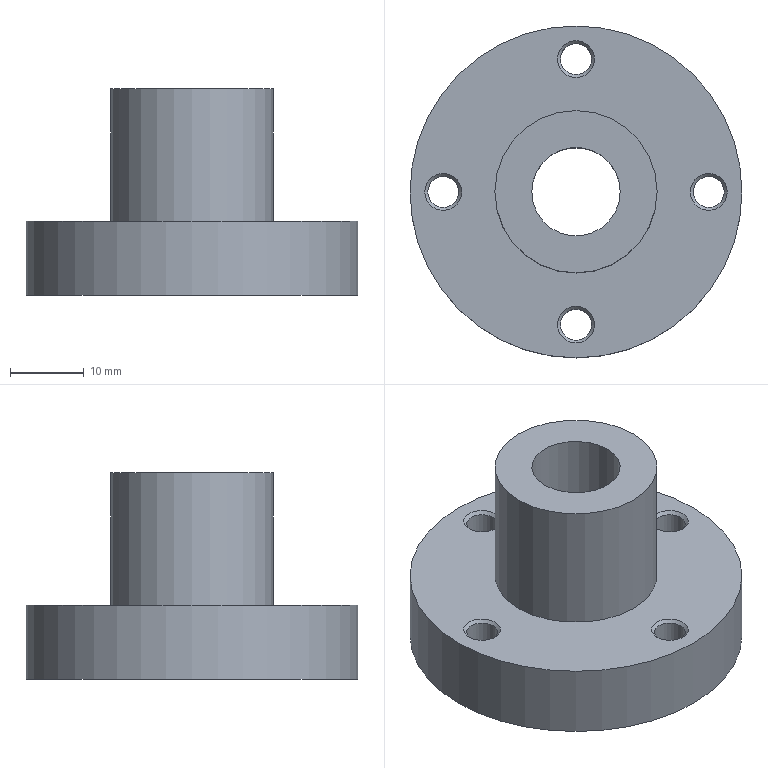Component | NX | GUIDE_SLEEVE | 1 solid | 18 faces | volume 19017 mm3 | cone 8 | cylinder 7 | plane 3 | commonest cylinder face diameters 4.2 x4 45 x1 22 x1 12 x1